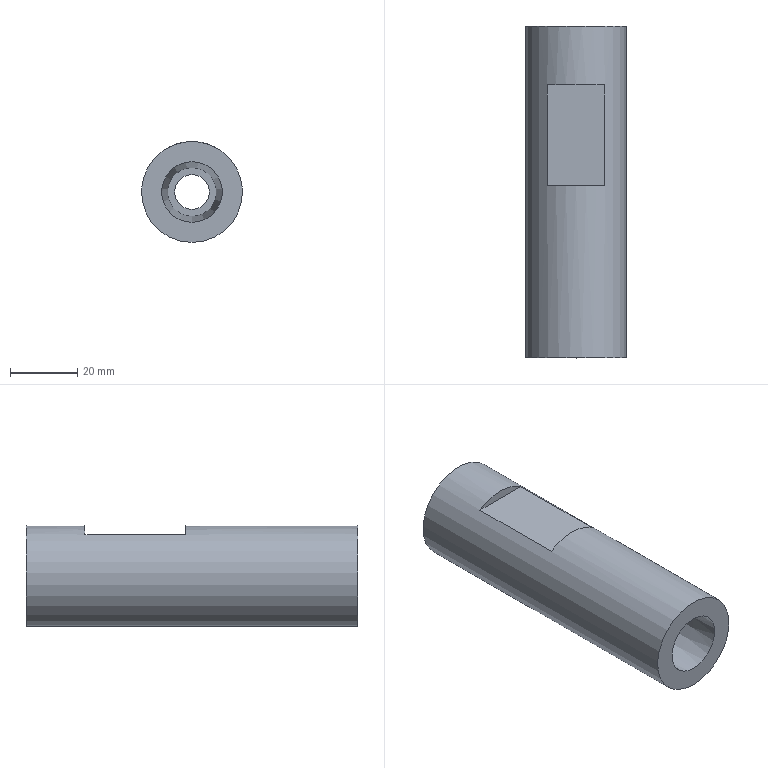Component | NX | SCREW_SLEEVE | 1 solid | 10 faces | box 30 x 98.6 x 30 mm | volume 51483 mm3 | plane 6 | cylinder 3 | cone 1 | commonest cylinder face diameters 14.5 x1 30 x1 10.3 x1
STEP:
#1=CARTESIAN_POINT('',(0.,0.,0.));
#2=DIRECTION('',(0.,0.,1.));
#3=DIRECTION('',(1.,0.,0.));
#4=AXIS2_PLACEMENT_3D('',#1,#2,#3);
#5=CARTESIAN_POINT('',(0.,-66.1,76.1));
#6=VERTEX_POINT('',#5);
#7=CARTESIAN_POINT('',(0.,-66.1,85.1));
#8=DIRECTION('',(0.,-1.,0.));
#9=DIRECTION('',(0.,0.,-1.));
#10=AXIS2_PLACEMENT_3D('',#7,#8,#9);
#11=CIRCLE('',#10,9.);
#12=CARTESIAN_POINT('',(0.,-66.1,100.1));
#13=DIRECTION('',(0.,1.,0.));
#14=DIRECTION('',(0.,0.,1.));
#15=AXIS2_PLACEMENT_3D('',#12,#13,#14);
#16=PLANE('',#15);
#17=CARTESIAN_POINT('',(-24.,0.));
#18=CARTESIAN_POINT('',(-24.,15.588));
#19=CARTESIAN_POINT('',(-10.5,7.794));
#20=CARTESIAN_POINT('',(3.,0.));
#21=CARTESIAN_POINT('',(-10.5,-7.794));
#22=CARTESIAN_POINT('',(-24.,-15.588));
#23=CARTESIAN_POINT('',(-24.,0.));
#24=(BOUNDED_CURVE()B_SPLINE_CURVE(2,(#17,#18,#19,#20,#21,#22,#23),.UNSPECIFIED.,.T.,.F.)B_SPLINE_CURVE_WITH_KNOTS((1,2,2,2,2,1),(-2.094,0.,2.094,4.189,6.283,8.378),.UNSPECIFIED.)CURVE()GEOMETRIC_REPRESENTATION_ITEM()RATIONAL_B_SPLINE_CURVE((1.,0.5,1.,0.5,1.,0.5,1.))REPRESENTATION_ITEM(''));
#25=(GEOMETRIC_REPRESENTATION_CONTEXT(2)PARAMETRIC_REPRESENTATION_CONTEXT()REPRESENTATION_CONTEXT('',''));
#26=DEFINITIONAL_REPRESENTATION('',(#24),#25);
#27=PCURVE('',#16,#26);
#28=CARTESIAN_POINT('',(0.,-66.1,85.1));
#29=DIRECTION('',(0.,-1.,0.));
#30=DIRECTION('',(0.,0.,-1.));
#31=AXIS2_PLACEMENT_3D('',#28,#29,#30);
#32=CONICAL_SURFACE('',#31,9.,0.02882);
#33=CARTESIAN_POINT('',(0.,0.));
#34=DIRECTION('',(1.,0.));
#35=VECTOR('',#34,1.);
#36=LINE('',#33,#35);
#37=(GEOMETRIC_REPRESENTATION_CONTEXT(2)PARAMETRIC_REPRESENTATION_CONTEXT()REPRESENTATION_CONTEXT('',''));
#38=DEFINITIONAL_REPRESENTATION('',(#36),#37);
#39=PCURVE('',#32,#38);
#40=SURFACE_CURVE('',#11,(#27,#39),.PCURVE_S1.);
#41=EDGE_CURVE('',#6,#6,#40,.T.);
#42=ORIENTED_EDGE('',*,*,#41,.F.);
#43=EDGE_LOOP('',(#42));
#44=FACE_BOUND('',#43,.T.);
#45=CARTESIAN_POINT('',(0.,-66.1,70.1));
#46=VERTEX_POINT('',#45);
#47=CARTESIAN_POINT('',(0.,-66.1,85.1));
#48=DIRECTION('',(0.,-1.,0.));
#49=DIRECTION('',(0.,0.,-1.));
#50=AXIS2_PLACEMENT_3D('',#47,#48,#49);
#51=CIRCLE('',#50,15.);
#52=CARTESIAN_POINT('',(-30.,0.));
#53=CARTESIAN_POINT('',(-30.,25.981));
#54=CARTESIAN_POINT('',(-7.5,12.99));
#55=CARTESIAN_POINT('',(15.,0.));
#56=CARTESIAN_POINT('',(-7.5,-12.99));
#57=CARTESIAN_POINT('',(-30.,-25.981));
#58=CARTESIAN_POINT('',(-30.,0.));
#59=(BOUNDED_CURVE()B_SPLINE_CURVE(2,(#52,#53,#54,#55,#56,#57,#58),.UNSPECIFIED.,.T.,.F.)B_SPLINE_CURVE_WITH_KNOTS((1,2,2,2,2,1),(-2.094,0.,2.094,4.189,6.283,8.378),.UNSPECIFIED.)CURVE()GEOMETRIC_REPRESENTATION_ITEM()RATIONAL_B_SPLINE_CURVE((1.,0.5,1.,0.5,1.,0.5,1.))REPRESENTATION_ITEM(''));
#60=(GEOMETRIC_REPRESENTATION_CONTEXT(2)PARAMETRIC_REPRESENTATION_CONTEXT()REPRESENTATION_CONTEXT('',''));
#61=DEFINITIONAL_REPRESENTATION('',(#59),#60);
#62=PCURVE('',#16,#61);
#63=CARTESIAN_POINT('',(0.,32.5,85.1));
#64=DIRECTION('',(0.,-1.,0.));
#65=DIRECTION('',(0.,0.,-1.));
#66=AXIS2_PLACEMENT_3D('',#63,#64,#65);
#67=CYLINDRICAL_SURFACE('',#66,15.);
#68=CARTESIAN_POINT('',(0.,98.6));
#69=DIRECTION('',(1.,0.));
#70=VECTOR('',#69,1.);
#71=LINE('',#68,#70);
#72=(GEOMETRIC_REPRESENTATION_CONTEXT(2)PARAMETRIC_REPRESENTATION_CONTEXT()REPRESENTATION_CONTEXT('',''));
#73=DEFINITIONAL_REPRESENTATION('',(#71),#72);
#74=PCURVE('',#67,#73);
#75=SURFACE_CURVE('',#51,(#62,#74),.PCURVE_S1.);
#76=EDGE_CURVE('',#46,#46,#75,.T.);
#77=ORIENTED_EDGE('',*,*,#76,.T.);
#78=EDGE_LOOP('',(#77));
#79=FACE_BOUND('',#78,.T.);
#80=ADVANCED_FACE('',(#44,#79),#16,.F.);
#81=CARTESIAN_POINT('',(0.,-5.4,77.85));
#82=VERTEX_POINT('',#81);
#83=CARTESIAN_POINT('',(0.,-5.4,85.1));
#84=DIRECTION('',(0.,-1.,0.));
#85=DIRECTION('',(0.,0.,-1.));
#86=AXIS2_PLACEMENT_3D('',#83,#84,#85);
#87=CIRCLE('',#86,7.25);
#88=CARTESIAN_POINT('',(0.,-60.7));
#89=DIRECTION('',(1.,0.));
#90=VECTOR('',#89,1.);
#91=LINE('',#88,#90);
#92=(GEOMETRIC_REPRESENTATION_CONTEXT(2)PARAMETRIC_REPRESENTATION_CONTEXT()REPRESENTATION_CONTEXT('',''));
#93=DEFINITIONAL_REPRESENTATION('',(#91),#92);
#94=PCURVE('',#32,#93);
#95=CARTESIAN_POINT('',(0.,32.5,85.1));
#96=DIRECTION('',(0.,-1.,0.));
#97=DIRECTION('',(0.,0.,-1.));
#98=AXIS2_PLACEMENT_3D('',#95,#96,#97);
#99=CYLINDRICAL_SURFACE('',#98,7.25);
#100=CARTESIAN_POINT('',(0.,37.9));
#101=DIRECTION('',(1.,0.));
#102=VECTOR('',#101,1.);
#103=LINE('',#100,#102);
#104=(GEOMETRIC_REPRESENTATION_CONTEXT(2)PARAMETRIC_REPRESENTATION_CONTEXT()REPRESENTATION_CONTEXT('',''));
#105=DEFINITIONAL_REPRESENTATION('',(#103),#104);
#106=PCURVE('',#99,#105);
#107=SURFACE_CURVE('',#87,(#94,#106),.PCURVE_S1.);
#108=EDGE_CURVE('',#82,#82,#107,.T.);
#109=ORIENTED_EDGE('',*,*,#108,.T.);
#110=CARTESIAN_POINT('',(0.,-5.4,77.85));
#111=CARTESIAN_POINT('',(0.,-66.1,76.1));
#112=B_SPLINE_CURVE_WITH_KNOTS('',1,(#110,#111),.UNSPECIFIED.,.F.,.F.,(2,2),(-60.725,0.),.PIECEWISE_BEZIER_KNOTS.);
#113=CARTESIAN_POINT('',(6.283,0.));
#114=DIRECTION('',(0.,1.));
#115=VECTOR('',#114,1.);
#116=LINE('',#113,#115);
#117=(GEOMETRIC_REPRESENTATION_CONTEXT(2)PARAMETRIC_REPRESENTATION_CONTEXT()REPRESENTATION_CONTEXT('',''));
#118=DEFINITIONAL_REPRESENTATION('',(#116),#117);
#119=PCURVE('',#32,#118);
#120=CARTESIAN_POINT('',(0.,0.));
#121=DIRECTION('',(0.,1.));
#122=VECTOR('',#121,1.);
#123=LINE('',#120,#122);
#124=(GEOMETRIC_REPRESENTATION_CONTEXT(2)PARAMETRIC_REPRESENTATION_CONTEXT()REPRESENTATION_CONTEXT('',''));
#125=DEFINITIONAL_REPRESENTATION('',(#123),#124);
#126=PCURVE('',#32,#125);
#127=SEAM_CURVE('',#112,(#119,#126),.PCURVE_S1.);
#128=EDGE_CURVE('',#82,#6,#127,.T.);
#129=ORIENTED_EDGE('',*,*,#128,.T.);
#130=ORIENTED_EDGE('',*,*,#41,.F.);
#131=ORIENTED_EDGE('',*,*,#128,.F.);
#132=EDGE_LOOP('',(#109,#129,#130,#131));
#133=FACE_BOUND('',#132,.F.);
#134=ADVANCED_FACE('',(#133),#32,.F.);
#135=CARTESIAN_POINT('',(0.,12.6,77.85));
#136=VERTEX_POINT('',#135);
#137=CARTESIAN_POINT('',(0.,12.6,85.1));
#138=DIRECTION('',(0.,-1.,0.));
#139=DIRECTION('',(0.,0.,-1.));
#140=AXIS2_PLACEMENT_3D('',#137,#138,#139);
#141=CIRCLE('',#140,7.25);
#142=CARTESIAN_POINT('',(0.,19.9));
#143=DIRECTION('',(1.,0.));
#144=VECTOR('',#143,1.);
#145=LINE('',#142,#144);
#146=(GEOMETRIC_REPRESENTATION_CONTEXT(2)PARAMETRIC_REPRESENTATION_CONTEXT()REPRESENTATION_CONTEXT('',''));
#147=DEFINITIONAL_REPRESENTATION('',(#145),#146);
#148=PCURVE('',#99,#147);
#149=CARTESIAN_POINT('',(0.,12.6,92.35));
#150=DIRECTION('',(0.,1.,0.));
#151=DIRECTION('',(0.,0.,1.));
#152=AXIS2_PLACEMENT_3D('',#149,#150,#151);
#153=PLANE('',#152);
#154=CARTESIAN_POINT('',(-14.5,0.));
#155=CARTESIAN_POINT('',(-14.5,12.557));
#156=CARTESIAN_POINT('',(-3.625,6.279));
#157=CARTESIAN_POINT('',(7.25,0.));
#158=CARTESIAN_POINT('',(-3.625,-6.279));
#159=CARTESIAN_POINT('',(-14.5,-12.557));
#160=CARTESIAN_POINT('',(-14.5,0.));
#161=(BOUNDED_CURVE()B_SPLINE_CURVE(2,(#154,#155,#156,#157,#158,#159,#160),.UNSPECIFIED.,.T.,.F.)B_SPLINE_CURVE_WITH_KNOTS((1,2,2,2,2,1),(-2.094,0.,2.094,4.189,6.283,8.378),.UNSPECIFIED.)CURVE()GEOMETRIC_REPRESENTATION_ITEM()RATIONAL_B_SPLINE_CURVE((1.,0.5,1.,0.5,1.,0.5,1.))REPRESENTATION_ITEM(''));
#162=(GEOMETRIC_REPRESENTATION_CONTEXT(2)PARAMETRIC_REPRESENTATION_CONTEXT()REPRESENTATION_CONTEXT('',''));
#163=DEFINITIONAL_REPRESENTATION('',(#161),#162);
#164=PCURVE('',#153,#163);
#165=SURFACE_CURVE('',#141,(#148,#164),.PCURVE_S1.);
#166=EDGE_CURVE('',#136,#136,#165,.T.);
#167=ORIENTED_EDGE('',*,*,#166,.T.);
#168=CARTESIAN_POINT('',(0.,12.6,77.85));
#169=CARTESIAN_POINT('',(0.,-5.4,77.85));
#170=B_SPLINE_CURVE_WITH_KNOTS('',1,(#168,#169),.UNSPECIFIED.,.F.,.F.,(2,2),(19.9,37.9),.PIECEWISE_BEZIER_KNOTS.);
#171=CARTESIAN_POINT('',(6.283,0.));
#172=DIRECTION('',(0.,1.));
#173=VECTOR('',#172,1.);
#174=LINE('',#171,#173);
#175=(GEOMETRIC_REPRESENTATION_CONTEXT(2)PARAMETRIC_REPRESENTATION_CONTEXT()REPRESENTATION_CONTEXT('',''));
#176=DEFINITIONAL_REPRESENTATION('',(#174),#175);
#177=PCURVE('',#99,#176);
#178=CARTESIAN_POINT('',(0.,0.));
#179=DIRECTION('',(0.,1.));
#180=VECTOR('',#179,1.);
#181=LINE('',#178,#180);
#182=(GEOMETRIC_REPRESENTATION_CONTEXT(2)PARAMETRIC_REPRESENTATION_CONTEXT()REPRESENTATION_CONTEXT('',''));
#183=DEFINITIONAL_REPRESENTATION('',(#181),#182);
#184=PCURVE('',#99,#183);
#185=SEAM_CURVE('',#170,(#177,#184),.PCURVE_S1.);
#186=EDGE_CURVE('',#136,#82,#185,.T.);
#187=ORIENTED_EDGE('',*,*,#186,.T.);
#188=ORIENTED_EDGE('',*,*,#108,.F.);
#189=ORIENTED_EDGE('',*,*,#186,.F.);
#190=EDGE_LOOP('',(#167,#187,#188,#189));
#191=FACE_BOUND('',#190,.F.);
#192=ADVANCED_FACE('',(#191),#99,.F.);
#193=CARTESIAN_POINT('',(0.,12.6,90.25));
#194=VERTEX_POINT('',#193);
#195=CARTESIAN_POINT('',(0.,12.6,79.95));
#196=VERTEX_POINT('',#195);
#197=CARTESIAN_POINT('',(0.,12.6,85.1));
#198=DIRECTION('',(0.,1.,0.));
#199=DIRECTION('',(0.,0.,1.));
#200=AXIS2_PLACEMENT_3D('',#197,#198,#199);
#201=CIRCLE('',#200,5.15);
#202=CARTESIAN_POINT('',(-7.25,0.));
#203=DIRECTION('',(1.,0.));
#204=AXIS2_PLACEMENT_2D('',#202,#203);
#205=CIRCLE('',#204,5.15);
#206=(GEOMETRIC_REPRESENTATION_CONTEXT(2)PARAMETRIC_REPRESENTATION_CONTEXT()REPRESENTATION_CONTEXT('',''));
#207=DEFINITIONAL_REPRESENTATION('',(#205),#206);
#208=PCURVE('',#153,#207);
#209=CARTESIAN_POINT('',(0.,32.5,85.1));
#210=DIRECTION('',(0.,-1.,0.));
#211=DIRECTION('',(0.,0.,-1.));
#212=AXIS2_PLACEMENT_3D('',#209,#210,#211);
#213=CYLINDRICAL_SURFACE('',#212,5.15);
#214=CARTESIAN_POINT('',(3.142,19.9));
#215=DIRECTION('',(-1.,0.));
#216=VECTOR('',#215,1.);
#217=LINE('',#214,#216);
#218=(GEOMETRIC_REPRESENTATION_CONTEXT(2)PARAMETRIC_REPRESENTATION_CONTEXT()REPRESENTATION_CONTEXT('',''));
#219=DEFINITIONAL_REPRESENTATION('',(#217),#218);
#220=PCURVE('',#213,#219);
#221=SURFACE_CURVE('',#201,(#208,#220),.PCURVE_S1.);
#222=EDGE_CURVE('',#194,#196,#221,.T.);
#223=ORIENTED_EDGE('',*,*,#222,.T.);
#224=CARTESIAN_POINT('',(0.,12.6,85.1));
#225=DIRECTION('',(0.,1.,0.));
#226=DIRECTION('',(0.,0.,1.));
#227=AXIS2_PLACEMENT_3D('',#224,#225,#226);
#228=CIRCLE('',#227,5.15);
#229=CARTESIAN_POINT('',(-7.25,0.));
#230=DIRECTION('',(1.,0.));
#231=AXIS2_PLACEMENT_2D('',#229,#230);
#232=CIRCLE('',#231,5.15);
#233=(GEOMETRIC_REPRESENTATION_CONTEXT(2)PARAMETRIC_REPRESENTATION_CONTEXT()REPRESENTATION_CONTEXT('',''));
#234=DEFINITIONAL_REPRESENTATION('',(#232),#233);
#235=PCURVE('',#153,#234);
#236=CARTESIAN_POINT('',(9.425,19.9));
#237=DIRECTION('',(-1.,0.));
#238=VECTOR('',#237,1.);
#239=LINE('',#236,#238);
#240=(GEOMETRIC_REPRESENTATION_CONTEXT(2)PARAMETRIC_REPRESENTATION_CONTEXT()REPRESENTATION_CONTEXT('',''));
#241=DEFINITIONAL_REPRESENTATION('',(#239),#240);
#242=PCURVE('',#213,#241);
#243=SURFACE_CURVE('',#228,(#235,#242),.PCURVE_S1.);
#244=EDGE_CURVE('',#196,#194,#243,.T.);
#245=ORIENTED_EDGE('',*,*,#244,.T.);
#246=EDGE_LOOP('',(#223,#245));
#247=FACE_BOUND('',#246,.T.);
#248=ORIENTED_EDGE('',*,*,#166,.T.);
#249=EDGE_LOOP('',(#248));
#250=FACE_BOUND('',#249,.T.);
#251=ADVANCED_FACE('',(#247,#250),#153,.F.);
#252=CARTESIAN_POINT('',(0.,32.5,79.95));
#253=VERTEX_POINT('',#252);
#254=CARTESIAN_POINT('',(0.,32.5,85.1));
#255=DIRECTION('',(0.,-1.,0.));
#256=DIRECTION('',(0.,0.,-1.));
#257=AXIS2_PLACEMENT_3D('',#254,#255,#256);
#258=CIRCLE('',#257,5.15);
#259=CARTESIAN_POINT('',(0.,32.5,90.1));
#260=DIRECTION('',(0.,-1.,0.));
#261=DIRECTION('',(0.,0.,-1.));
#262=AXIS2_PLACEMENT_3D('',#259,#260,#261);
#263=PLANE('',#262);
#264=CARTESIAN_POINT('',(5.,0.));
#265=DIRECTION('',(1.,0.));
#266=AXIS2_PLACEMENT_2D('',#264,#265);
#267=CIRCLE('',#266,5.15);
#268=(GEOMETRIC_REPRESENTATION_CONTEXT(2)PARAMETRIC_REPRESENTATION_CONTEXT()REPRESENTATION_CONTEXT('',''));
#269=DEFINITIONAL_REPRESENTATION('',(#267),#268);
#270=PCURVE('',#263,#269);
#271=CARTESIAN_POINT('',(0.,0.));
#272=DIRECTION('',(1.,0.));
#273=VECTOR('',#272,1.);
#274=LINE('',#271,#273);
#275=(GEOMETRIC_REPRESENTATION_CONTEXT(2)PARAMETRIC_REPRESENTATION_CONTEXT()REPRESENTATION_CONTEXT('',''));
#276=DEFINITIONAL_REPRESENTATION('',(#274),#275);
#277=PCURVE('',#213,#276);
#278=SURFACE_CURVE('',#258,(#270,#277),.PCURVE_S1.);
#279=EDGE_CURVE('',#253,#253,#278,.T.);
#280=ORIENTED_EDGE('',*,*,#279,.T.);
#281=EDGE_LOOP('',(#280));
#282=FACE_BOUND('',#281,.T.);
#283=CARTESIAN_POINT('',(0.,32.5,70.1));
#284=VERTEX_POINT('',#283);
#285=CARTESIAN_POINT('',(0.,32.5,85.1));
#286=DIRECTION('',(0.,-1.,0.));
#287=DIRECTION('',(0.,0.,-1.));
#288=AXIS2_PLACEMENT_3D('',#285,#286,#287);
#289=CIRCLE('',#288,15.);
#290=CARTESIAN_POINT('',(5.,0.));
#291=DIRECTION('',(1.,0.));
#292=AXIS2_PLACEMENT_2D('',#290,#291);
#293=CIRCLE('',#292,15.);
#294=(GEOMETRIC_REPRESENTATION_CONTEXT(2)PARAMETRIC_REPRESENTATION_CONTEXT()REPRESENTATION_CONTEXT('',''));
#295=DEFINITIONAL_REPRESENTATION('',(#293),#294);
#296=PCURVE('',#263,#295);
#297=CARTESIAN_POINT('',(0.,0.));
#298=DIRECTION('',(1.,0.));
#299=VECTOR('',#298,1.);
#300=LINE('',#297,#299);
#301=(GEOMETRIC_REPRESENTATION_CONTEXT(2)PARAMETRIC_REPRESENTATION_CONTEXT()REPRESENTATION_CONTEXT('',''));
#302=DEFINITIONAL_REPRESENTATION('',(#300),#301);
#303=PCURVE('',#67,#302);
#304=SURFACE_CURVE('',#289,(#296,#303),.PCURVE_S1.);
#305=EDGE_CURVE('',#284,#284,#304,.T.);
#306=ORIENTED_EDGE('',*,*,#305,.F.);
#307=EDGE_LOOP('',(#306));
#308=FACE_BOUND('',#307,.T.);
#309=ADVANCED_FACE('',(#282,#308),#263,.F.);
#310=ORIENTED_EDGE('',*,*,#76,.F.);
#311=CARTESIAN_POINT('',(-0.,32.5,70.1));
#312=CARTESIAN_POINT('',(-0.,-66.1,70.1));
#313=B_SPLINE_CURVE_WITH_KNOTS('',1,(#311,#312),.UNSPECIFIED.,.F.,.F.,(2,2),(0.,98.6),.PIECEWISE_BEZIER_KNOTS.);
#314=CARTESIAN_POINT('',(0.,0.));
#315=DIRECTION('',(0.,1.));
#316=VECTOR('',#315,1.);
#317=LINE('',#314,#316);
#318=(GEOMETRIC_REPRESENTATION_CONTEXT(2)PARAMETRIC_REPRESENTATION_CONTEXT()REPRESENTATION_CONTEXT('',''));
#319=DEFINITIONAL_REPRESENTATION('',(#317),#318);
#320=PCURVE('',#67,#319);
#321=CARTESIAN_POINT('',(6.283,0.));
#322=DIRECTION('',(0.,1.));
#323=VECTOR('',#322,1.);
#324=LINE('',#321,#323);
#325=(GEOMETRIC_REPRESENTATION_CONTEXT(2)PARAMETRIC_REPRESENTATION_CONTEXT()REPRESENTATION_CONTEXT('',''));
#326=DEFINITIONAL_REPRESENTATION('',(#324),#325);
#327=PCURVE('',#67,#326);
#328=SEAM_CURVE('',#313,(#320,#327),.PCURVE_S1.);
#329=EDGE_CURVE('',#284,#46,#328,.T.);
#330=ORIENTED_EDGE('',*,*,#329,.F.);
#331=ORIENTED_EDGE('',*,*,#305,.T.);
#332=ORIENTED_EDGE('',*,*,#329,.T.);
#333=EDGE_LOOP('',(#310,#330,#331,#332));
#334=FACE_BOUND('',#333,.T.);
#335=CARTESIAN_POINT('',(8.585,15.,97.4));
#336=VERTEX_POINT('',#335);
#337=CARTESIAN_POINT('',(8.585,-15.,97.4));
#338=VERTEX_POINT('',#337);
#339=CARTESIAN_POINT('',(8.585,32.5,97.4));
#340=DIRECTION('',(0.,-1.,0.));
#341=VECTOR('',#340,1.);
#342=LINE('',#339,#341);
#343=CARTESIAN_POINT('',(2.532,0.));
#344=DIRECTION('',(0.,1.));
#345=VECTOR('',#344,1.);
#346=LINE('',#343,#345);
#347=(GEOMETRIC_REPRESENTATION_CONTEXT(2)PARAMETRIC_REPRESENTATION_CONTEXT()REPRESENTATION_CONTEXT('',''));
#348=DEFINITIONAL_REPRESENTATION('',(#346),#347);
#349=PCURVE('',#67,#348);
#350=CARTESIAN_POINT('',(-20.,-15.,97.4));
#351=DIRECTION('',(0.,0.,-1.));
#352=DIRECTION('',(0.,1.,0.));
#353=AXIS2_PLACEMENT_3D('',#350,#351,#352);
#354=PLANE('',#353);
#355=CARTESIAN_POINT('',(47.5,28.585));
#356=DIRECTION('',(-1.,0.));
#357=VECTOR('',#356,1.);
#358=LINE('',#355,#357);
#359=(GEOMETRIC_REPRESENTATION_CONTEXT(2)PARAMETRIC_REPRESENTATION_CONTEXT()REPRESENTATION_CONTEXT('',''));
#360=DEFINITIONAL_REPRESENTATION('',(#358),#359);
#361=PCURVE('',#354,#360);
#362=SURFACE_CURVE('',#342,(#349,#361),.PCURVE_S1.);
#363=EDGE_CURVE('',#336,#338,#362,.T.);
#364=ORIENTED_EDGE('',*,*,#363,.T.);
#365=CARTESIAN_POINT('',(-8.585,-15.,97.4));
#366=VERTEX_POINT('',#365);
#367=CARTESIAN_POINT('',(0.,-15.,85.1));
#368=DIRECTION('',(0.,-1.,-0.));
#369=DIRECTION('',(0.,0.,-1.));
#370=AXIS2_PLACEMENT_3D('',#367,#368,#369);
#371=CIRCLE('',#370,15.);
#372=CARTESIAN_POINT('',(-0.,47.5));
#373=DIRECTION('',(1.,0.));
#374=VECTOR('',#373,1.);
#375=LINE('',#372,#374);
#376=(GEOMETRIC_REPRESENTATION_CONTEXT(2)PARAMETRIC_REPRESENTATION_CONTEXT()REPRESENTATION_CONTEXT('',''));
#377=DEFINITIONAL_REPRESENTATION('',(#375),#376);
#378=PCURVE('',#67,#377);
#379=CARTESIAN_POINT('',(-20.,-15.,112.4));
#380=DIRECTION('',(0.,-1.,-0.));
#381=DIRECTION('',(0.,0.,-1.));
#382=AXIS2_PLACEMENT_3D('',#379,#380,#381);
#383=PLANE('',#382);
#384=CARTESIAN_POINT('',(27.3,20.));
#385=DIRECTION('',(1.,0.));
#386=AXIS2_PLACEMENT_2D('',#384,#385);
#387=CIRCLE('',#386,15.);
#388=(GEOMETRIC_REPRESENTATION_CONTEXT(2)PARAMETRIC_REPRESENTATION_CONTEXT()REPRESENTATION_CONTEXT('',''));
#389=DEFINITIONAL_REPRESENTATION('',(#387),#388);
#390=PCURVE('',#383,#389);
#391=SURFACE_CURVE('',#371,(#378,#390),.PCURVE_S1.);
#392=EDGE_CURVE('',#338,#366,#391,.T.);
#393=ORIENTED_EDGE('',*,*,#392,.T.);
#394=CARTESIAN_POINT('',(-8.585,15.,97.4));
#395=VERTEX_POINT('',#394);
#396=CARTESIAN_POINT('',(-8.585,32.5,97.4));
#397=DIRECTION('',(0.,1.,0.));
#398=VECTOR('',#397,1.);
#399=LINE('',#396,#398);
#400=CARTESIAN_POINT('',(3.751,0.));
#401=DIRECTION('',(0.,-1.));
#402=VECTOR('',#401,1.);
#403=LINE('',#400,#402);
#404=(GEOMETRIC_REPRESENTATION_CONTEXT(2)PARAMETRIC_REPRESENTATION_CONTEXT()REPRESENTATION_CONTEXT('',''));
#405=DEFINITIONAL_REPRESENTATION('',(#403),#404);
#406=PCURVE('',#67,#405);
#407=CARTESIAN_POINT('',(47.5,11.415));
#408=DIRECTION('',(1.,0.));
#409=VECTOR('',#408,1.);
#410=LINE('',#407,#409);
#411=(GEOMETRIC_REPRESENTATION_CONTEXT(2)PARAMETRIC_REPRESENTATION_CONTEXT()REPRESENTATION_CONTEXT('',''));
#412=DEFINITIONAL_REPRESENTATION('',(#410),#411);
#413=PCURVE('',#354,#412);
#414=SURFACE_CURVE('',#399,(#406,#413),.PCURVE_S1.);
#415=EDGE_CURVE('',#366,#395,#414,.T.);
#416=ORIENTED_EDGE('',*,*,#415,.T.);
#417=CARTESIAN_POINT('',(0.,15.,85.1));
#418=DIRECTION('',(0.,1.,0.));
#419=DIRECTION('',(0.,-0.,1.));
#420=AXIS2_PLACEMENT_3D('',#417,#418,#419);
#421=CIRCLE('',#420,15.);
#422=CARTESIAN_POINT('',(9.425,17.5));
#423=DIRECTION('',(-1.,0.));
#424=VECTOR('',#423,1.);
#425=LINE('',#422,#424);
#426=(GEOMETRIC_REPRESENTATION_CONTEXT(2)PARAMETRIC_REPRESENTATION_CONTEXT()REPRESENTATION_CONTEXT('',''));
#427=DEFINITIONAL_REPRESENTATION('',(#425),#426);
#428=PCURVE('',#67,#427);
#429=CARTESIAN_POINT('',(-20.,15.,97.4));
#430=DIRECTION('',(0.,1.,0.));
#431=DIRECTION('',(0.,-0.,1.));
#432=AXIS2_PLACEMENT_3D('',#429,#430,#431);
#433=PLANE('',#432);
#434=CARTESIAN_POINT('',(-12.3,20.));
#435=DIRECTION('',(1.,0.));
#436=AXIS2_PLACEMENT_2D('',#434,#435);
#437=CIRCLE('',#436,15.);
#438=(GEOMETRIC_REPRESENTATION_CONTEXT(2)PARAMETRIC_REPRESENTATION_CONTEXT()REPRESENTATION_CONTEXT('',''));
#439=DEFINITIONAL_REPRESENTATION('',(#437),#438);
#440=PCURVE('',#433,#439);
#441=SURFACE_CURVE('',#421,(#428,#440),.PCURVE_S1.);
#442=EDGE_CURVE('',#395,#336,#441,.T.);
#443=ORIENTED_EDGE('',*,*,#442,.T.);
#444=EDGE_LOOP('',(#364,#393,#416,#443));
#445=FACE_BOUND('',#444,.T.);
#446=ADVANCED_FACE('',(#334,#445),#67,.T.);
#447=CARTESIAN_POINT('',(-20.,-15.,97.4));
#448=DIRECTION('',(-1.,0.,0.));
#449=VECTOR('',#448,1.);
#450=LINE('',#447,#449);
#451=CARTESIAN_POINT('',(15.,0.));
#452=DIRECTION('',(0.,-1.));
#453=VECTOR('',#452,1.);
#454=LINE('',#451,#453);
#455=(GEOMETRIC_REPRESENTATION_CONTEXT(2)PARAMETRIC_REPRESENTATION_CONTEXT()REPRESENTATION_CONTEXT('',''));
#456=DEFINITIONAL_REPRESENTATION('',(#454),#455);
#457=PCURVE('',#383,#456);
#458=CARTESIAN_POINT('',(0.,0.));
#459=DIRECTION('',(0.,-1.));
#460=VECTOR('',#459,1.);
#461=LINE('',#458,#460);
#462=(GEOMETRIC_REPRESENTATION_CONTEXT(2)PARAMETRIC_REPRESENTATION_CONTEXT()REPRESENTATION_CONTEXT('',''));
#463=DEFINITIONAL_REPRESENTATION('',(#461),#462);
#464=PCURVE('',#354,#463);
#465=SURFACE_CURVE('',#450,(#457,#464),.PCURVE_S1.);
#466=EDGE_CURVE('',#338,#366,#465,.T.);
#467=ORIENTED_EDGE('',*,*,#466,.T.);
#468=ORIENTED_EDGE('',*,*,#392,.F.);
#469=EDGE_LOOP('',(#467,#468));
#470=FACE_BOUND('',#469,.T.);
#471=ADVANCED_FACE('',(#470),#383,.F.);
#472=CARTESIAN_POINT('',(-20.,15.,97.4));
#473=DIRECTION('',(-1.,0.,0.));
#474=VECTOR('',#473,1.);
#475=LINE('',#472,#474);
#476=CARTESIAN_POINT('',(30.,0.));
#477=DIRECTION('',(0.,-1.));
#478=VECTOR('',#477,1.);
#479=LINE('',#476,#478);
#480=(GEOMETRIC_REPRESENTATION_CONTEXT(2)PARAMETRIC_REPRESENTATION_CONTEXT()REPRESENTATION_CONTEXT('',''));
#481=DEFINITIONAL_REPRESENTATION('',(#479),#480);
#482=PCURVE('',#354,#481);
#483=CARTESIAN_POINT('',(0.,0.));
#484=DIRECTION('',(0.,-1.));
#485=VECTOR('',#484,1.);
#486=LINE('',#483,#485);
#487=(GEOMETRIC_REPRESENTATION_CONTEXT(2)PARAMETRIC_REPRESENTATION_CONTEXT()REPRESENTATION_CONTEXT('',''));
#488=DEFINITIONAL_REPRESENTATION('',(#486),#487);
#489=PCURVE('',#433,#488);
#490=SURFACE_CURVE('',#475,(#482,#489),.PCURVE_S1.);
#491=EDGE_CURVE('',#336,#395,#490,.T.);
#492=ORIENTED_EDGE('',*,*,#491,.T.);
#493=ORIENTED_EDGE('',*,*,#415,.F.);
#494=ORIENTED_EDGE('',*,*,#466,.F.);
#495=ORIENTED_EDGE('',*,*,#363,.F.);
#496=EDGE_LOOP('',(#492,#493,#494,#495));
#497=FACE_BOUND('',#496,.T.);
#498=ADVANCED_FACE('',(#497),#354,.F.);
#499=ORIENTED_EDGE('',*,*,#491,.F.);
#500=ORIENTED_EDGE('',*,*,#442,.F.);
#501=EDGE_LOOP('',(#499,#500));
#502=FACE_BOUND('',#501,.T.);
#503=ADVANCED_FACE('',(#502),#433,.F.);
#504=ORIENTED_EDGE('',*,*,#279,.T.);
#505=CARTESIAN_POINT('',(0.,32.5,79.95));
#506=CARTESIAN_POINT('',(0.,12.6,79.95));
#507=B_SPLINE_CURVE_WITH_KNOTS('',1,(#505,#506),.UNSPECIFIED.,.F.,.F.,(2,2),(0.,19.9),.PIECEWISE_BEZIER_KNOTS.);
#508=CARTESIAN_POINT('',(6.283,0.));
#509=DIRECTION('',(0.,1.));
#510=VECTOR('',#509,1.);
#511=LINE('',#508,#510);
#512=(GEOMETRIC_REPRESENTATION_CONTEXT(2)PARAMETRIC_REPRESENTATION_CONTEXT()REPRESENTATION_CONTEXT('',''));
#513=DEFINITIONAL_REPRESENTATION('',(#511),#512);
#514=PCURVE('',#213,#513);
#515=CARTESIAN_POINT('',(0.,0.));
#516=DIRECTION('',(0.,1.));
#517=VECTOR('',#516,1.);
#518=LINE('',#515,#517);
#519=(GEOMETRIC_REPRESENTATION_CONTEXT(2)PARAMETRIC_REPRESENTATION_CONTEXT()REPRESENTATION_CONTEXT('',''));
#520=DEFINITIONAL_REPRESENTATION('',(#518),#519);
#521=PCURVE('',#213,#520);
#522=SEAM_CURVE('',#507,(#514,#521),.PCURVE_S1.);
#523=EDGE_CURVE('',#253,#196,#522,.T.);
#524=ORIENTED_EDGE('',*,*,#523,.T.);
#525=ORIENTED_EDGE('',*,*,#244,.T.);
#526=ORIENTED_EDGE('',*,*,#222,.T.);
#527=ORIENTED_EDGE('',*,*,#523,.F.);
#528=EDGE_LOOP('',(#504,#524,#525,#526,#527));
#529=FACE_BOUND('',#528,.F.);
#530=ADVANCED_FACE('',(#529),#213,.F.);
#531=CLOSED_SHELL('',(#80,#134,#192,#251,#309,#446,#471,#498,#503,#530));
#532=MANIFOLD_SOLID_BREP('',#531);
#533=(LENGTH_UNIT()NAMED_UNIT(*)SI_UNIT(.MILLI.,.METRE.));
#534=UNCERTAINTY_MEASURE_WITH_UNIT(LENGTH_MEASURE(0.000005),#533,'','');
#535=(NAMED_UNIT(*)PLANE_ANGLE_UNIT()SI_UNIT($,.RADIAN.));
#536=(NAMED_UNIT(*)SI_UNIT($,.STERADIAN.)SOLID_ANGLE_UNIT());
#537=(GEOMETRIC_REPRESENTATION_CONTEXT(3)GLOBAL_UNCERTAINTY_ASSIGNED_CONTEXT((#534))GLOBAL_UNIT_ASSIGNED_CONTEXT((#533,#535,#536))REPRESENTATION_CONTEXT('',''));
#538=ADVANCED_BREP_SHAPE_REPRESENTATION('',(#4,#532),#537);